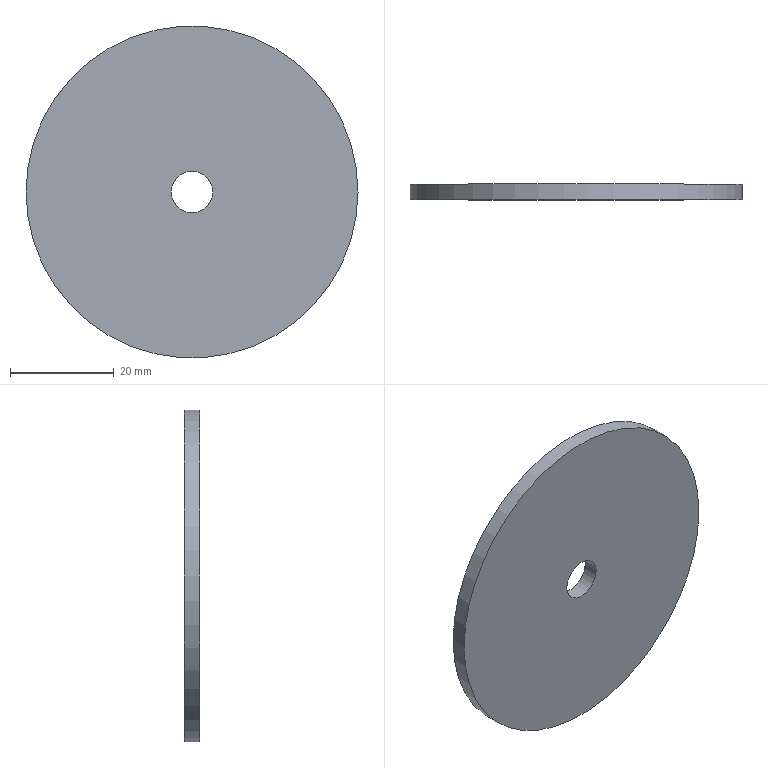Component | NX | BASE_CIRCLE | 1 solid | 4 faces | box 64 x 3 x 64 mm | volume 9500 mm3 | cylinder 2 | plane 2 | commonest cylinder face diameters 64 x1 8 x1
STEP:
#1=CARTESIAN_POINT('',(0.,0.,0.));
#2=DIRECTION('',(0.,0.,1.));
#3=DIRECTION('',(1.,0.,0.));
#4=AXIS2_PLACEMENT_3D('',#1,#2,#3);
#5=CARTESIAN_POINT('',(-165.451,-31.96,29.835));
#6=VERTEX_POINT('',#5);
#7=CARTESIAN_POINT('',(-133.451,-31.96,29.835));
#8=DIRECTION('',(0.,1.,0.));
#9=DIRECTION('',(-1.,0.,-0.));
#10=AXIS2_PLACEMENT_3D('',#7,#8,#9);
#11=CIRCLE('',#10,32.);
#12=CARTESIAN_POINT('',(-133.451,-31.96,29.835));
#13=DIRECTION('',(0.,-1.,0.));
#14=DIRECTION('',(0.,0.,1.));
#15=AXIS2_PLACEMENT_3D('',#12,#13,#14);
#16=CYLINDRICAL_SURFACE('',#15,32.);
#17=CARTESIAN_POINT('',(7.854,0.));
#18=DIRECTION('',(-1.,0.));
#19=VECTOR('',#18,1.);
#20=LINE('',#17,#19);
#21=(GEOMETRIC_REPRESENTATION_CONTEXT(2)PARAMETRIC_REPRESENTATION_CONTEXT()REPRESENTATION_CONTEXT('',''));
#22=DEFINITIONAL_REPRESENTATION('',(#20),#21);
#23=PCURVE('',#16,#22);
#24=CARTESIAN_POINT('',(-133.451,-31.96,29.835));
#25=DIRECTION('',(0.,1.,0.));
#26=DIRECTION('',(0.,0.,-1.));
#27=AXIS2_PLACEMENT_3D('',#24,#25,#26);
#28=PLANE('',#27);
#29=CARTESIAN_POINT('',(0.,0.));
#30=DIRECTION('',(0.,1.));
#31=AXIS2_PLACEMENT_2D('',#29,#30);
#32=CIRCLE('',#31,32.);
#33=(GEOMETRIC_REPRESENTATION_CONTEXT(2)PARAMETRIC_REPRESENTATION_CONTEXT()REPRESENTATION_CONTEXT('',''));
#34=DEFINITIONAL_REPRESENTATION('',(#32),#33);
#35=PCURVE('',#28,#34);
#36=SURFACE_CURVE('',#11,(#23,#35),.PCURVE_S1.);
#37=EDGE_CURVE('',#6,#6,#36,.T.);
#38=ORIENTED_EDGE('',*,*,#37,.F.);
#39=CARTESIAN_POINT('',(-165.451,-34.96,29.835));
#40=VERTEX_POINT('',#39);
#41=CARTESIAN_POINT('',(-165.451,-31.96,29.835));
#42=CARTESIAN_POINT('',(-165.451,-34.96,29.835));
#43=B_SPLINE_CURVE_WITH_KNOTS('',1,(#41,#42),.UNSPECIFIED.,.F.,.F.,(2,2),(0.,3.),.PIECEWISE_BEZIER_KNOTS.);
#44=CARTESIAN_POINT('',(7.854,0.));
#45=DIRECTION('',(0.,1.));
#46=VECTOR('',#45,1.);
#47=LINE('',#44,#46);
#48=(GEOMETRIC_REPRESENTATION_CONTEXT(2)PARAMETRIC_REPRESENTATION_CONTEXT()REPRESENTATION_CONTEXT('',''));
#49=DEFINITIONAL_REPRESENTATION('',(#47),#48);
#50=PCURVE('',#16,#49);
#51=CARTESIAN_POINT('',(1.571,0.));
#52=DIRECTION('',(0.,1.));
#53=VECTOR('',#52,1.);
#54=LINE('',#51,#53);
#55=(GEOMETRIC_REPRESENTATION_CONTEXT(2)PARAMETRIC_REPRESENTATION_CONTEXT()REPRESENTATION_CONTEXT('',''));
#56=DEFINITIONAL_REPRESENTATION('',(#54),#55);
#57=PCURVE('',#16,#56);
#58=SEAM_CURVE('',#43,(#50,#57),.PCURVE_S1.);
#59=EDGE_CURVE('',#6,#40,#58,.T.);
#60=ORIENTED_EDGE('',*,*,#59,.T.);
#61=CARTESIAN_POINT('',(-133.451,-34.96,29.835));
#62=DIRECTION('',(0.,1.,0.));
#63=DIRECTION('',(-1.,0.,-0.));
#64=AXIS2_PLACEMENT_3D('',#61,#62,#63);
#65=CIRCLE('',#64,32.);
#66=CARTESIAN_POINT('',(7.854,3.));
#67=DIRECTION('',(-1.,0.));
#68=VECTOR('',#67,1.);
#69=LINE('',#66,#68);
#70=(GEOMETRIC_REPRESENTATION_CONTEXT(2)PARAMETRIC_REPRESENTATION_CONTEXT()REPRESENTATION_CONTEXT('',''));
#71=DEFINITIONAL_REPRESENTATION('',(#69),#70);
#72=PCURVE('',#16,#71);
#73=CARTESIAN_POINT('',(-133.451,-34.96,29.835));
#74=DIRECTION('',(0.,1.,0.));
#75=DIRECTION('',(0.,0.,-1.));
#76=AXIS2_PLACEMENT_3D('',#73,#74,#75);
#77=PLANE('',#76);
#78=CARTESIAN_POINT('',(0.,0.));
#79=DIRECTION('',(0.,1.));
#80=AXIS2_PLACEMENT_2D('',#78,#79);
#81=CIRCLE('',#80,32.);
#82=(GEOMETRIC_REPRESENTATION_CONTEXT(2)PARAMETRIC_REPRESENTATION_CONTEXT()REPRESENTATION_CONTEXT('',''));
#83=DEFINITIONAL_REPRESENTATION('',(#81),#82);
#84=PCURVE('',#77,#83);
#85=SURFACE_CURVE('',#65,(#72,#84),.PCURVE_S1.);
#86=EDGE_CURVE('',#40,#40,#85,.T.);
#87=ORIENTED_EDGE('',*,*,#86,.T.);
#88=ORIENTED_EDGE('',*,*,#59,.F.);
#89=EDGE_LOOP('',(#38,#60,#87,#88));
#90=FACE_BOUND('',#89,.T.);
#91=ADVANCED_FACE('',(#90),#16,.T.);
#92=CARTESIAN_POINT('',(-137.451,-31.96,29.835));
#93=VERTEX_POINT('',#92);
#94=CARTESIAN_POINT('',(-133.451,-31.96,29.835));
#95=DIRECTION('',(0.,1.,0.));
#96=DIRECTION('',(-1.,0.,0.));
#97=AXIS2_PLACEMENT_3D('',#94,#95,#96);
#98=CIRCLE('',#97,4.);
#99=CARTESIAN_POINT('',(-133.451,-31.96,29.835));
#100=DIRECTION('',(0.,-1.,0.));
#101=DIRECTION('',(0.,0.,1.));
#102=AXIS2_PLACEMENT_3D('',#99,#100,#101);
#103=CYLINDRICAL_SURFACE('',#102,4.);
#104=CARTESIAN_POINT('',(7.854,0.));
#105=DIRECTION('',(-1.,0.));
#106=VECTOR('',#105,1.);
#107=LINE('',#104,#106);
#108=(GEOMETRIC_REPRESENTATION_CONTEXT(2)PARAMETRIC_REPRESENTATION_CONTEXT()REPRESENTATION_CONTEXT('',''));
#109=DEFINITIONAL_REPRESENTATION('',(#107),#108);
#110=PCURVE('',#103,#109);
#111=CARTESIAN_POINT('',(0.,0.));
#112=DIRECTION('',(0.,1.));
#113=AXIS2_PLACEMENT_2D('',#111,#112);
#114=CIRCLE('',#113,4.);
#115=(GEOMETRIC_REPRESENTATION_CONTEXT(2)PARAMETRIC_REPRESENTATION_CONTEXT()REPRESENTATION_CONTEXT('',''));
#116=DEFINITIONAL_REPRESENTATION('',(#114),#115);
#117=PCURVE('',#28,#116);
#118=SURFACE_CURVE('',#98,(#110,#117),.PCURVE_S1.);
#119=EDGE_CURVE('',#93,#93,#118,.T.);
#120=ORIENTED_EDGE('',*,*,#119,.F.);
#121=CARTESIAN_POINT('',(-137.451,-34.96,29.835));
#122=VERTEX_POINT('',#121);
#123=CARTESIAN_POINT('',(-137.451,-31.96,29.835));
#124=CARTESIAN_POINT('',(-137.451,-34.96,29.835));
#125=B_SPLINE_CURVE_WITH_KNOTS('',1,(#123,#124),.UNSPECIFIED.,.F.,.F.,(2,2),(0.,3.),.PIECEWISE_BEZIER_KNOTS.);
#126=CARTESIAN_POINT('',(7.854,0.));
#127=DIRECTION('',(0.,1.));
#128=VECTOR('',#127,1.);
#129=LINE('',#126,#128);
#130=(GEOMETRIC_REPRESENTATION_CONTEXT(2)PARAMETRIC_REPRESENTATION_CONTEXT()REPRESENTATION_CONTEXT('',''));
#131=DEFINITIONAL_REPRESENTATION('',(#129),#130);
#132=PCURVE('',#103,#131);
#133=CARTESIAN_POINT('',(1.571,0.));
#134=DIRECTION('',(0.,1.));
#135=VECTOR('',#134,1.);
#136=LINE('',#133,#135);
#137=(GEOMETRIC_REPRESENTATION_CONTEXT(2)PARAMETRIC_REPRESENTATION_CONTEXT()REPRESENTATION_CONTEXT('',''));
#138=DEFINITIONAL_REPRESENTATION('',(#136),#137);
#139=PCURVE('',#103,#138);
#140=SEAM_CURVE('',#125,(#132,#139),.PCURVE_S1.);
#141=EDGE_CURVE('',#93,#122,#140,.T.);
#142=ORIENTED_EDGE('',*,*,#141,.T.);
#143=CARTESIAN_POINT('',(-133.451,-34.96,29.835));
#144=DIRECTION('',(0.,1.,0.));
#145=DIRECTION('',(-1.,0.,0.));
#146=AXIS2_PLACEMENT_3D('',#143,#144,#145);
#147=CIRCLE('',#146,4.);
#148=CARTESIAN_POINT('',(7.854,3.));
#149=DIRECTION('',(-1.,0.));
#150=VECTOR('',#149,1.);
#151=LINE('',#148,#150);
#152=(GEOMETRIC_REPRESENTATION_CONTEXT(2)PARAMETRIC_REPRESENTATION_CONTEXT()REPRESENTATION_CONTEXT('',''));
#153=DEFINITIONAL_REPRESENTATION('',(#151),#152);
#154=PCURVE('',#103,#153);
#155=CARTESIAN_POINT('',(0.,0.));
#156=DIRECTION('',(0.,1.));
#157=AXIS2_PLACEMENT_2D('',#155,#156);
#158=CIRCLE('',#157,4.);
#159=(GEOMETRIC_REPRESENTATION_CONTEXT(2)PARAMETRIC_REPRESENTATION_CONTEXT()REPRESENTATION_CONTEXT('',''));
#160=DEFINITIONAL_REPRESENTATION('',(#158),#159);
#161=PCURVE('',#77,#160);
#162=SURFACE_CURVE('',#147,(#154,#161),.PCURVE_S1.);
#163=EDGE_CURVE('',#122,#122,#162,.T.);
#164=ORIENTED_EDGE('',*,*,#163,.T.);
#165=ORIENTED_EDGE('',*,*,#141,.F.);
#166=EDGE_LOOP('',(#120,#142,#164,#165));
#167=FACE_BOUND('',#166,.F.);
#168=ADVANCED_FACE('',(#167),#103,.F.);
#169=ORIENTED_EDGE('',*,*,#37,.T.);
#170=EDGE_LOOP('',(#169));
#171=FACE_BOUND('',#170,.T.);
#172=ORIENTED_EDGE('',*,*,#119,.F.);
#173=EDGE_LOOP('',(#172));
#174=FACE_BOUND('',#173,.T.);
#175=ADVANCED_FACE('',(#171,#174),#28,.T.);
#176=ORIENTED_EDGE('',*,*,#86,.F.);
#177=EDGE_LOOP('',(#176));
#178=FACE_BOUND('',#177,.T.);
#179=ORIENTED_EDGE('',*,*,#163,.T.);
#180=EDGE_LOOP('',(#179));
#181=FACE_BOUND('',#180,.T.);
#182=ADVANCED_FACE('',(#178,#181),#77,.F.);
#183=CLOSED_SHELL('',(#91,#168,#175,#182));
#184=MANIFOLD_SOLID_BREP('',#183);
#185=(LENGTH_UNIT()NAMED_UNIT(*)SI_UNIT(.MILLI.,.METRE.));
#186=UNCERTAINTY_MEASURE_WITH_UNIT(LENGTH_MEASURE(0.00001),#185,'','');
#187=(NAMED_UNIT(*)PLANE_ANGLE_UNIT()SI_UNIT($,.RADIAN.));
#188=(NAMED_UNIT(*)SI_UNIT($,.STERADIAN.)SOLID_ANGLE_UNIT());
#189=(GEOMETRIC_REPRESENTATION_CONTEXT(3)GLOBAL_UNCERTAINTY_ASSIGNED_CONTEXT((#186))GLOBAL_UNIT_ASSIGNED_CONTEXT((#185,#187,#188))REPRESENTATION_CONTEXT('',''));
#190=ADVANCED_BREP_SHAPE_REPRESENTATION('',(#4,#184),#189);